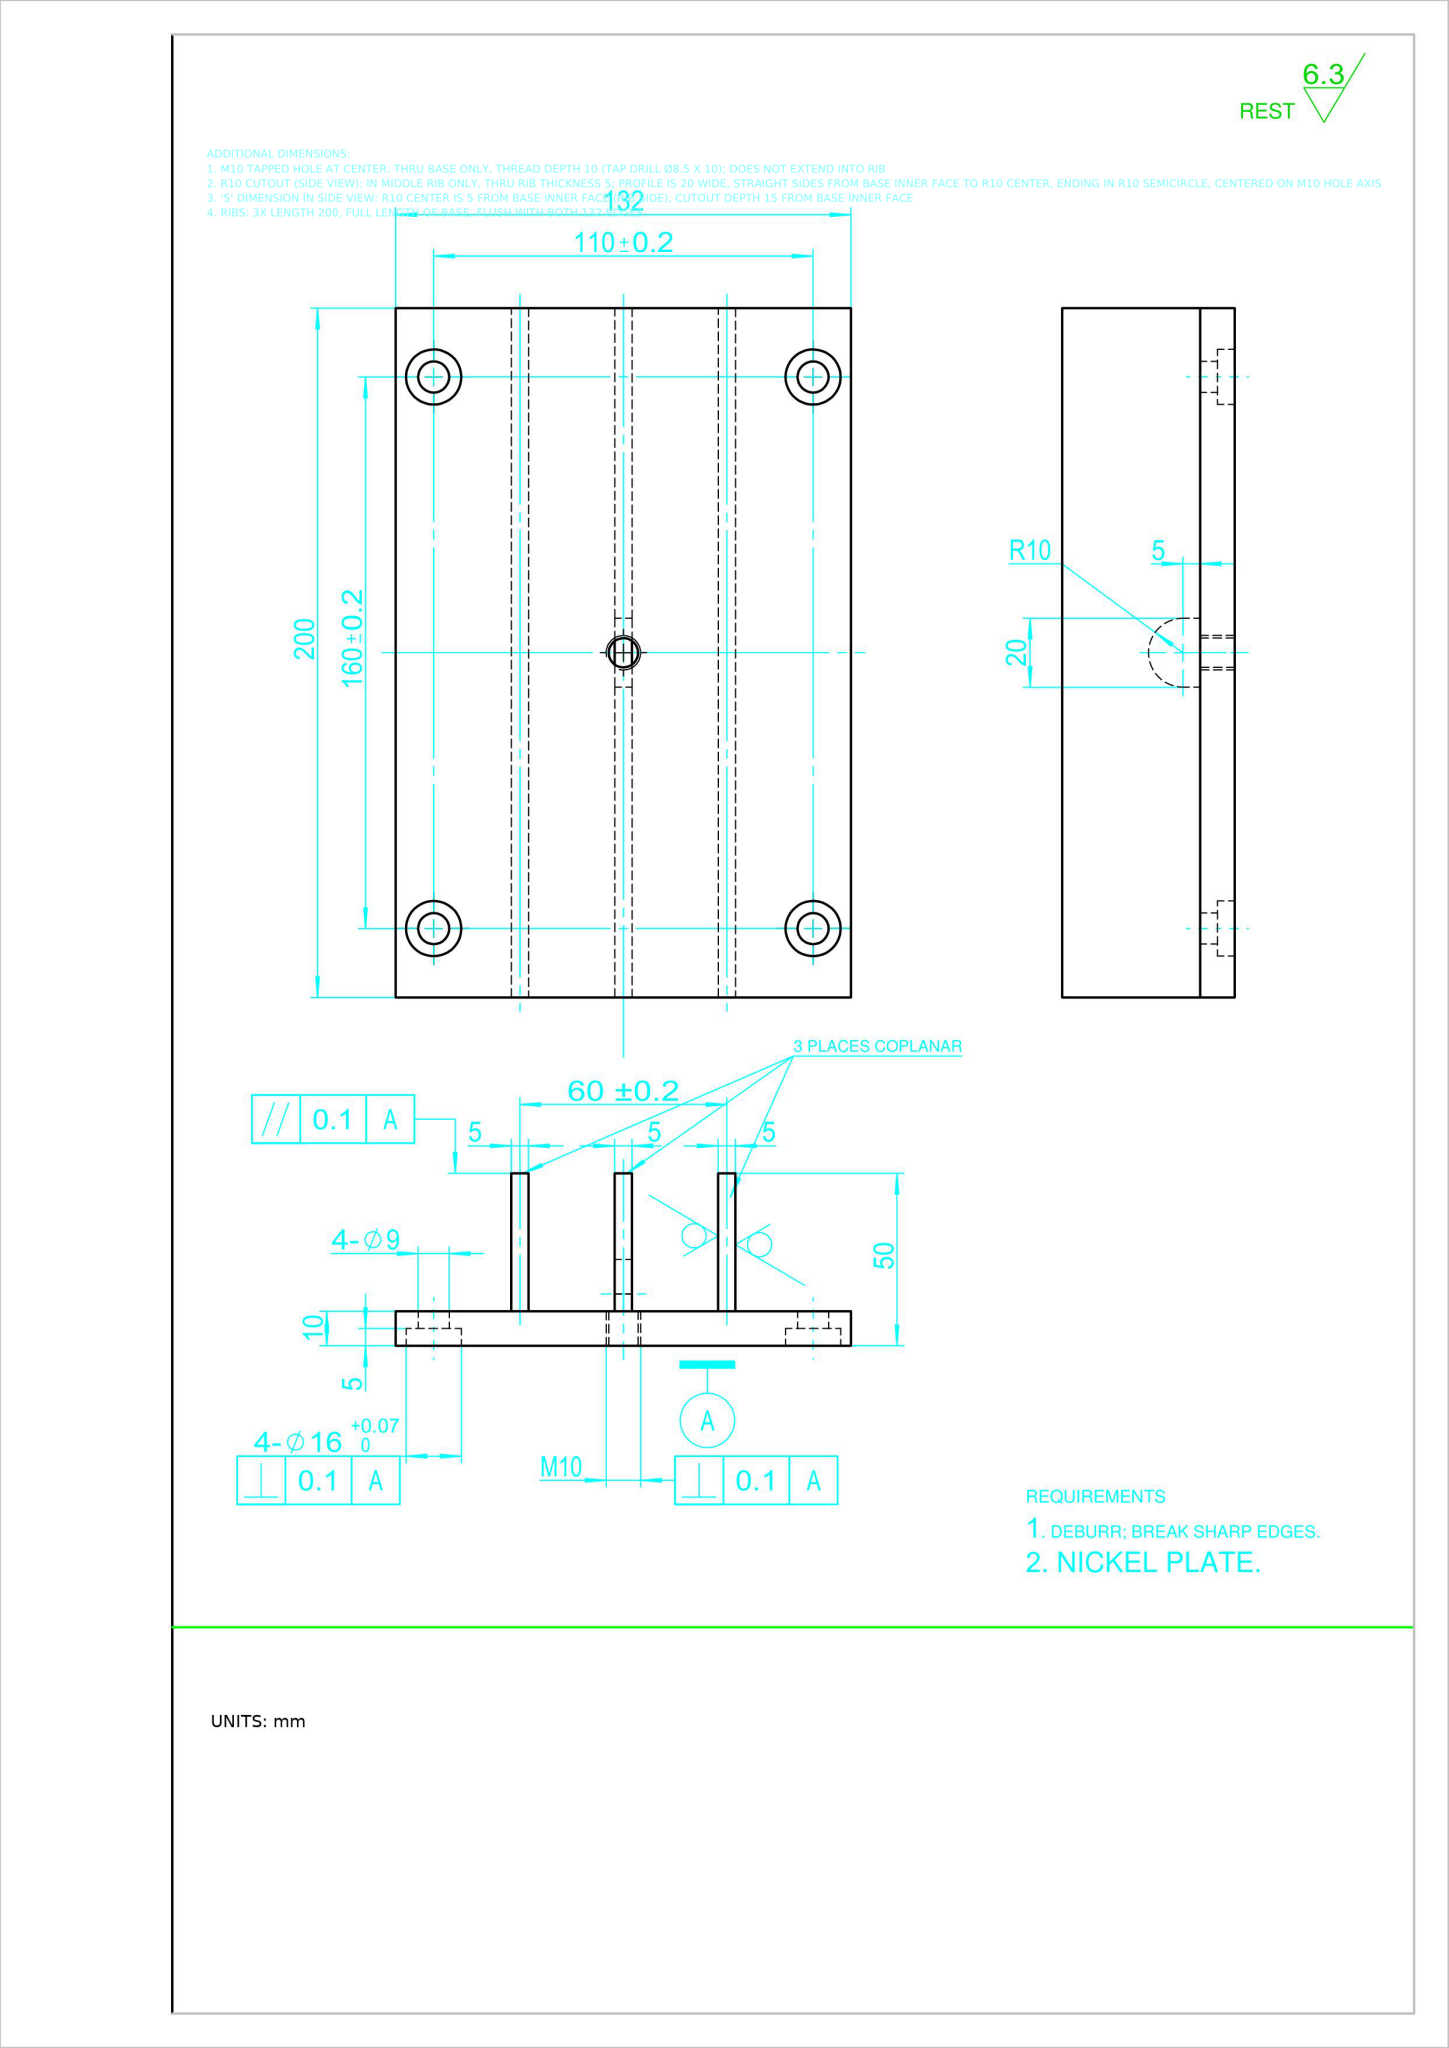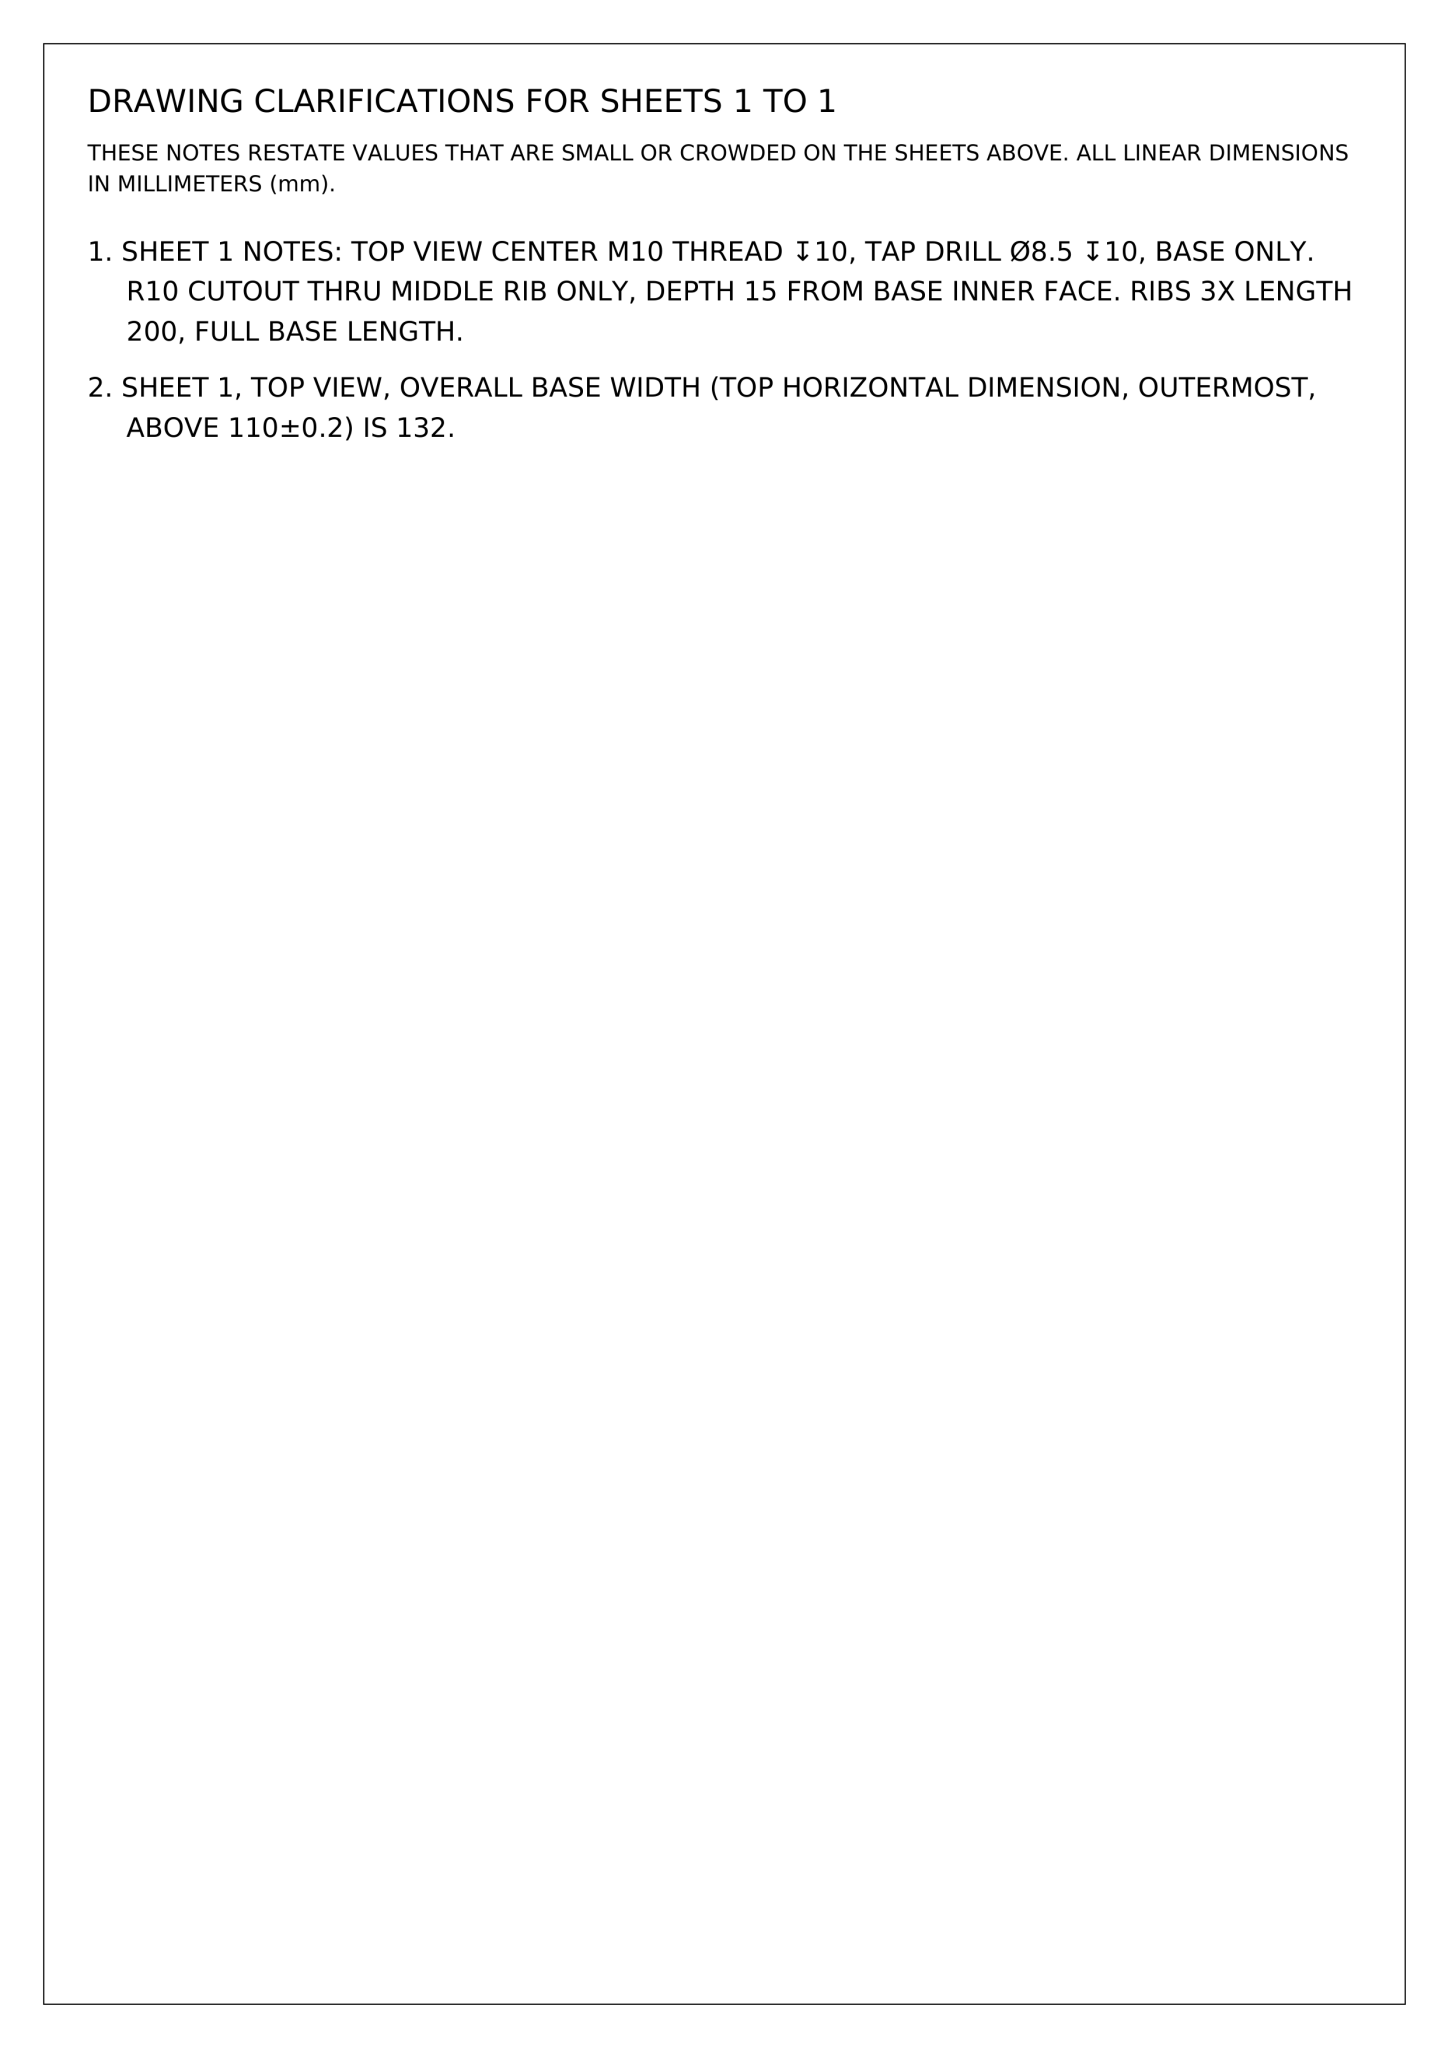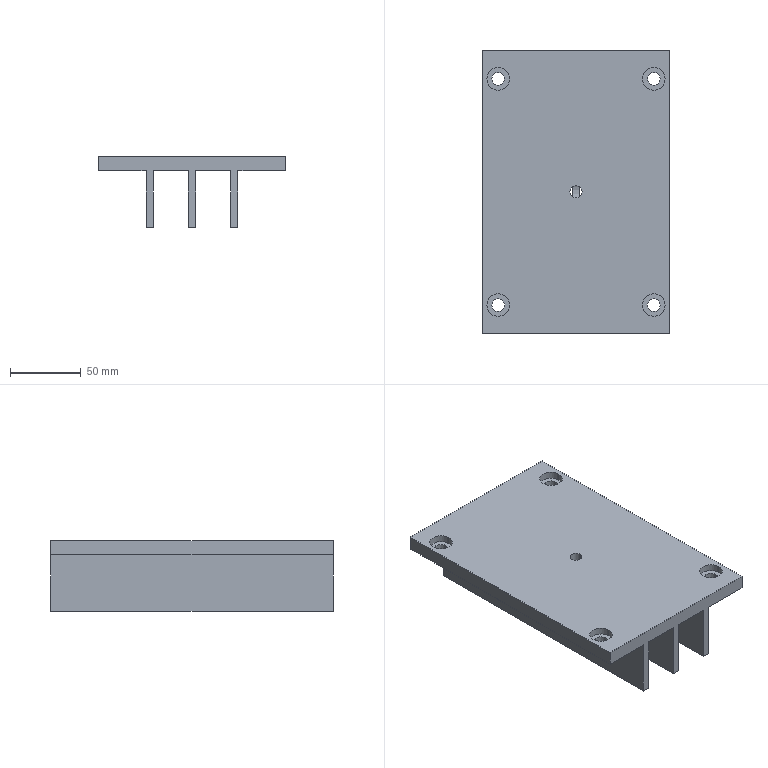Part | NX | mm | 1 solid | 42 faces | box 132 x 200 x 50 mm | volume 376854 mm3 | plane 23 | cylinder 19 | commonest cylinder face diameters 9 x8 16 x8 8.5 x2 20 x1